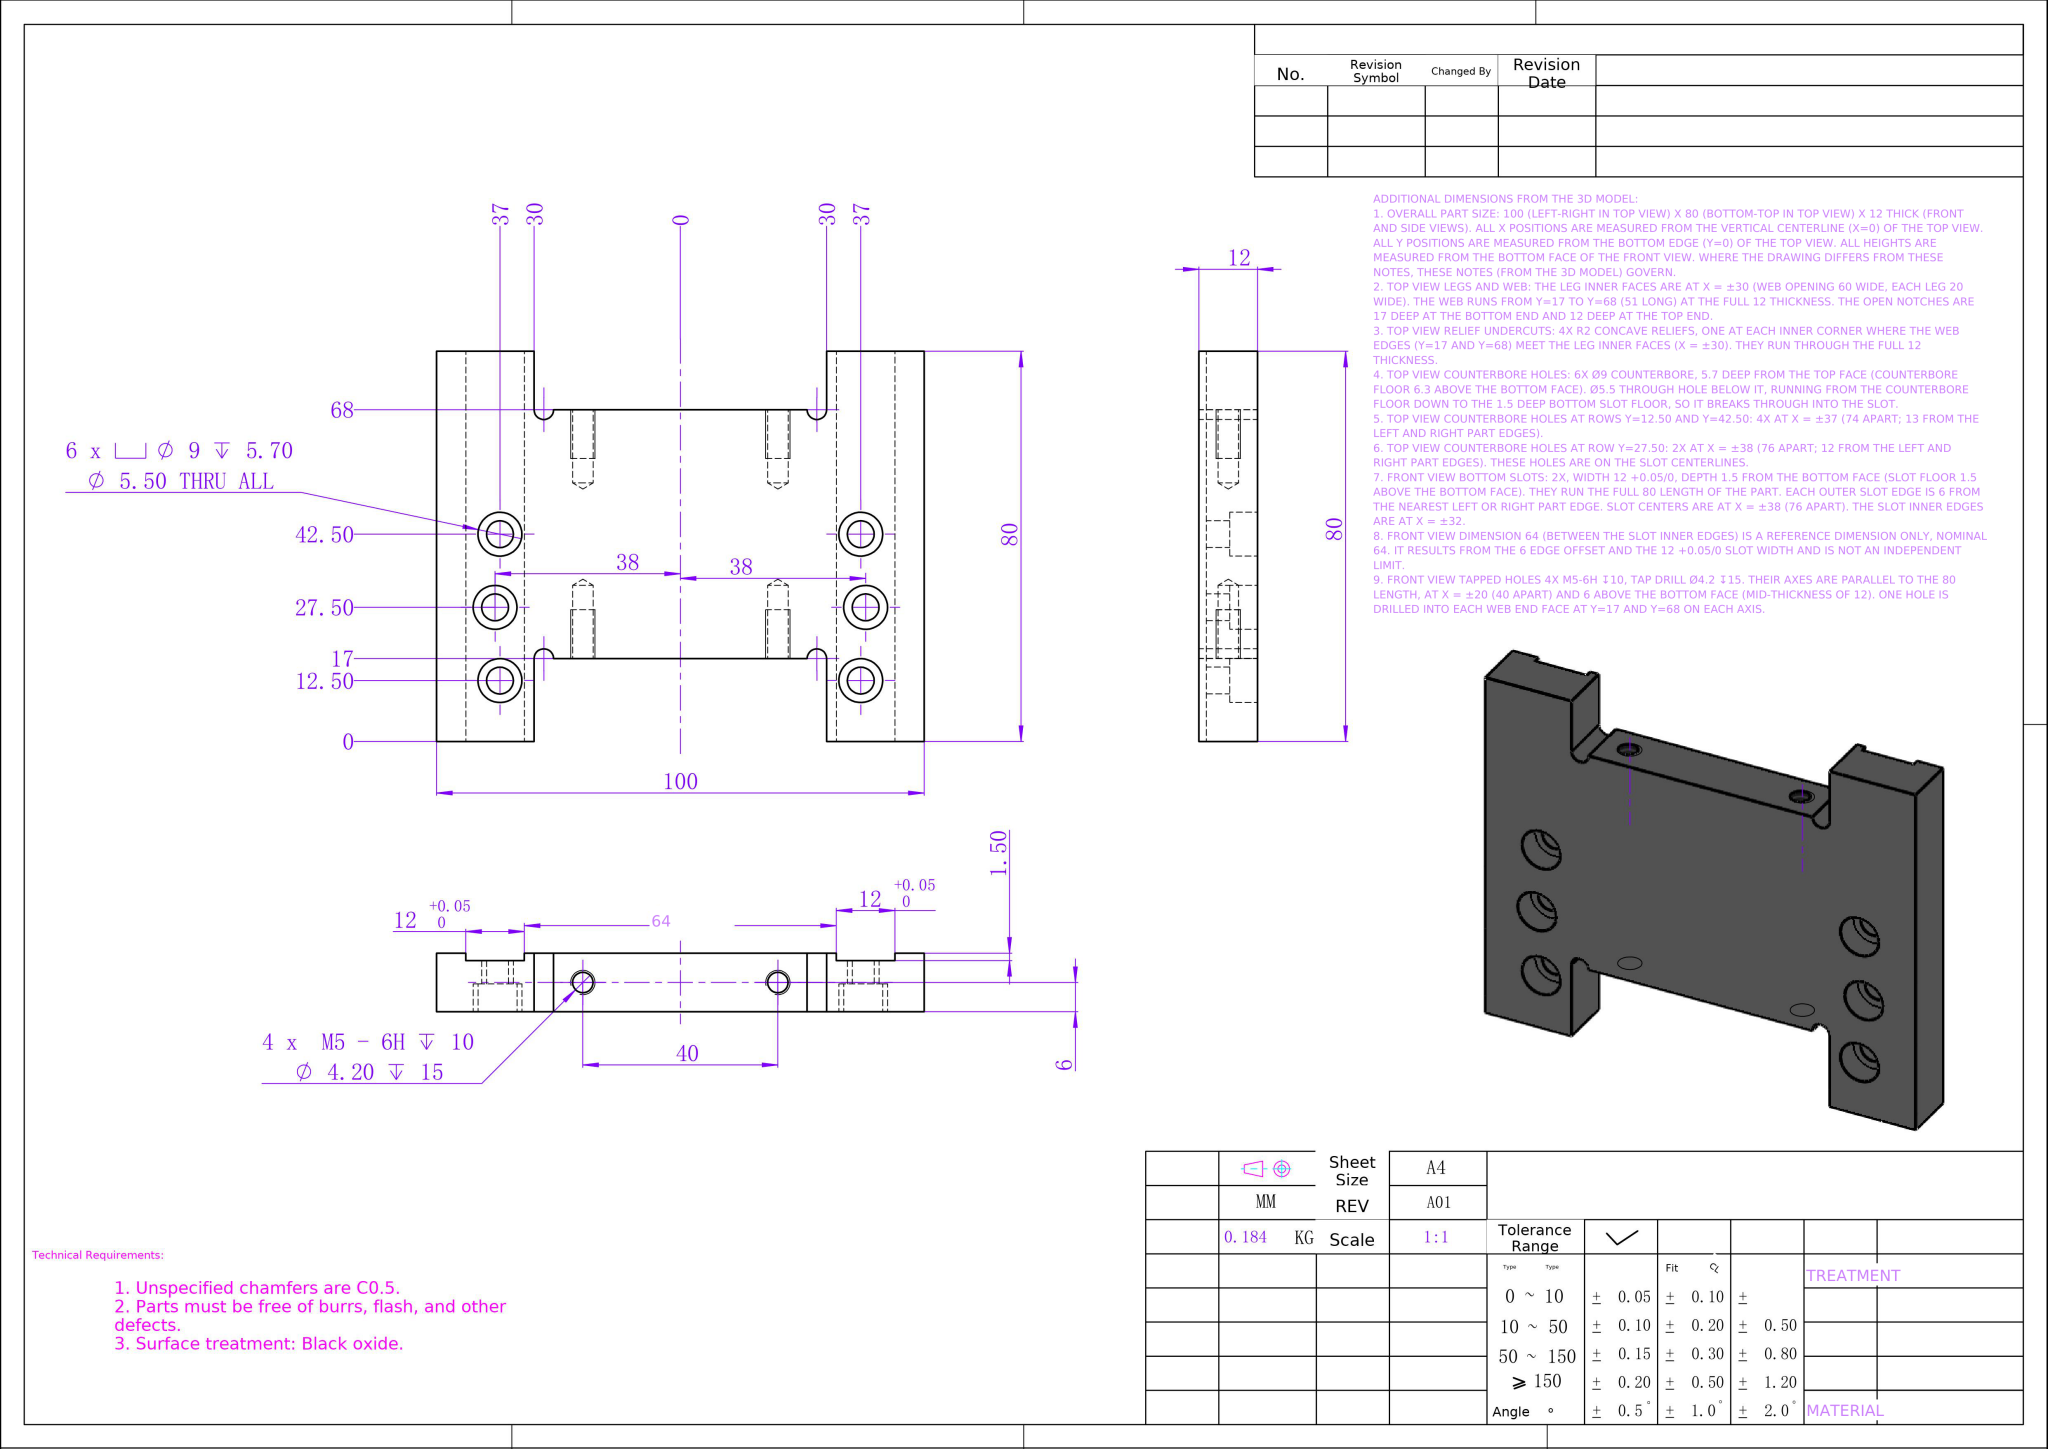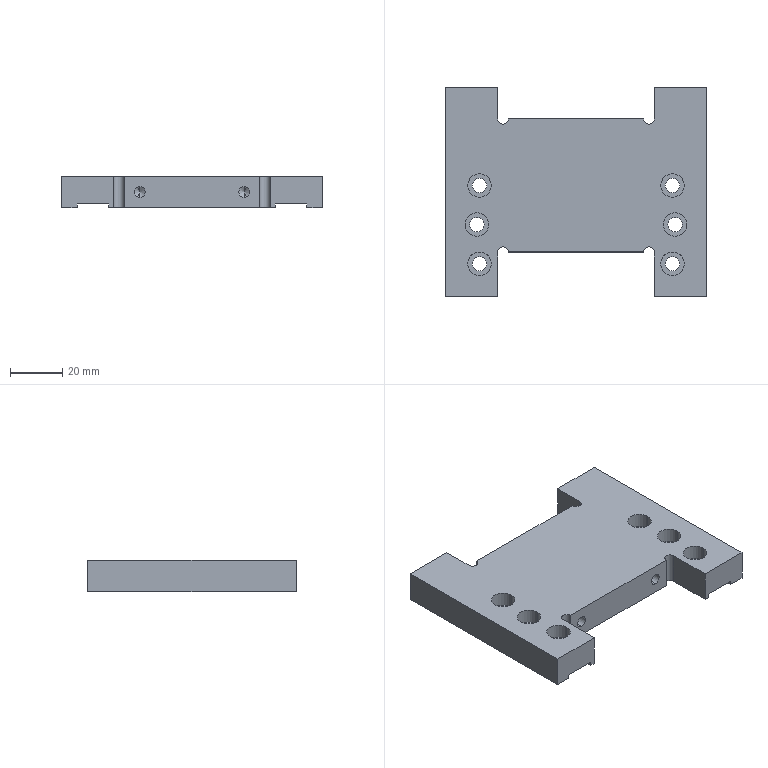Part | NX | mm | 1 solid | 72 faces | box 100 x 80 x 12 mm | volume 68224 mm3 | cylinder 36 | plane 28 | cone 8 | commonest cylinder face diameters 5.5 x12 9 x12 4.2 x8 4 x4